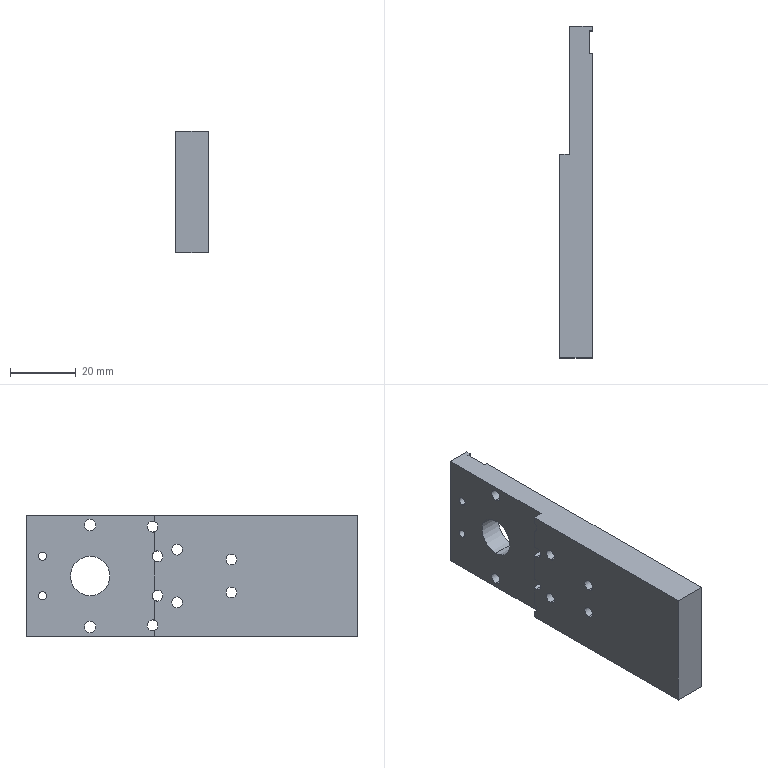Component | SolidWorks | AS-011-JG0136-1 | 1 solid | 42 faces | box 10 x 101 x 37 mm | volume 31155 mm3 | cylinder 26 | plane 16 | commonest cylinder face diameters 3.3 x16 2.5 x4 3.5 x4 12 x2
build123d program:
from build123d import *

# Parameters (mm, degrees)
SKETCH1_W           = 37
SKETCH1_H           = 101
SKETCH1_R           = 6
SKETCH1_R_2         = 1.75
SKETCH1_R_3         = 1.65
SKETCH1_R_4         = 1.25
BOSS_EXTRUDE1_DEPTH = 10
SKETCH6_OUTSIDE_W   = 33.606
SKETCH6_OUTSIDE_H   = 124.606
CUT_EXTRUDE1_DEPTH  = 109.028


with BuildPart() as part:
    # Sketch1 → Boss-Extrude1 (new body)
    with BuildSketch(Plane.XY):
        with Locations((18.5, 50.5)):
            Rectangle(SKETCH1_W, SKETCH1_H)
        with Locations((18.5, 81.5)):
            Circle(SKETCH1_R, mode=Mode.SUBTRACT)
        with Locations((3, 81.5)):
            Circle(SKETCH1_R_2, mode=Mode.SUBTRACT)
        with Locations((34, 81.5)):
            Circle(SKETCH1_R_2, mode=Mode.SUBTRACT)
        with Locations((12.5, 61)):
            Circle(SKETCH1_R_3, mode=Mode.SUBTRACT)
        with Locations((24.5, 61)):
            Circle(SKETCH1_R_3, mode=Mode.SUBTRACT)
        with Locations((10.5, 55)):
            Circle(SKETCH1_R_3, mode=Mode.SUBTRACT)
        with Locations((26.5, 55)):
            Circle(SKETCH1_R_3, mode=Mode.SUBTRACT)
        with Locations((13.5, 38.5)):
            Circle(SKETCH1_R_3, mode=Mode.SUBTRACT)
        with Locations((23.5, 38.5)):
            Circle(SKETCH1_R_3, mode=Mode.SUBTRACT)
        with Locations((12.5, 96)):
            Circle(SKETCH1_R_4, mode=Mode.SUBTRACT)
        with Locations((24.5, 96)):
            Circle(SKETCH1_R_4, mode=Mode.SUBTRACT)
        with Locations((3.5, 62.5)):
            Circle(SKETCH1_R_3, mode=Mode.SUBTRACT)
        with Locations((33.5, 62.5)):
            Circle(SKETCH1_R_3, mode=Mode.SUBTRACT)
    extrude(amount=-BOSS_EXTRUDE1_DEPTH)

    # Sketch6 outside → Cut-Extrude1 (cut, through all)
    with BuildSketch(Plane.ZY):
        with Locations((-5, 50.5)):
            Rectangle(SKETCH6_OUTSIDE_W, SKETCH6_OUTSIDE_H)
        Polygon((-7, 101), (-7, 62), (-10, 62), (-10, 0), (0, 0), (0, 92.5), (-1, 92.5), (-1, 99.5), (0, 99.5), (0, 101), align=None, mode=Mode.SUBTRACT)
    extrude(amount=-CUT_EXTRUDE1_DEPTH, mode=Mode.SUBTRACT)


solid = part.part

# Placed as in the assembly
solid = solid.moved(Location((-30, -99.5, 8.5), (0, 90, 0)))